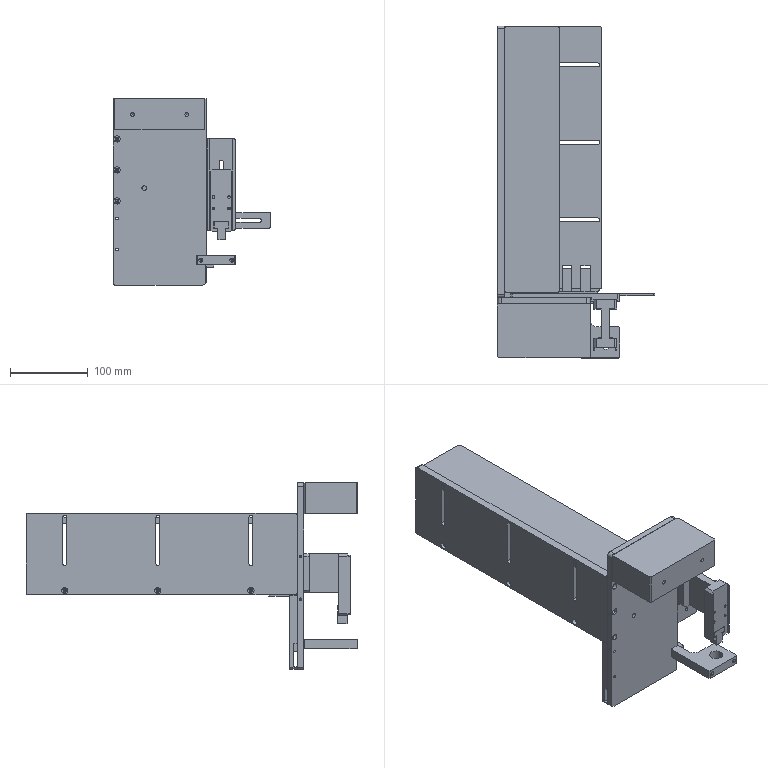Assembly | SolidWorks | mm | 13 component files | 13 solids | 410 faces | box 203.38 x 428 x 240 mm | volume 1719772 mm3 | plane 202 | cylinder 160 | cone 48 | commonest cylinder face diameters 5 x25 4.2 x20 3.3 x20 6 x16 8 x16 4.5 x16 4 x13 5.5 x10
Bill of materials:
SecondGenerationFour-sidedLabelingFeedingAdjustmentBaffle | 1 |  | Thin rectangular base plate with rounded corners carrying three evenly spaced rectangular ribs/blocks standing across its width; one block has a small cross hole in its end face.
SecondGenerationFour-sidedLabelingFeedingCylinderConnector | 1 |  | T-shaped block: wider rectangular head over a narrower rectangular stem, with a round through hole running vertically through the center.
SecondGenerationFour-sidedLabelingFeedingFrontBaffle | 1 |  | Long thin rectangular plate with three narrow slots running across its width, open at one long edge, plus a comb-like set of rectangular notches/fingers at one end; a small hole or slot is visible on one end edge.
SecondGenerationFour-sidedLabelingFeedingFrontLimitPlate | 1 |  | Long, slender rectangular bar with a shallow step at one end and a downturned rectangular block at the other end, forming an L/hook shape in side profile; a round hole goes through the end block.
SecondGenerationFour-sidedLabelingFeedingLimitPlate | 1 |  | Elongated rectangular bar with two round holes along its length and a reduced-thickness notched section near one end that ends in a small hook/lip.
SecondGenerationFour-sidedLabelingFeedingRearBaffle | 1 |  | Long thin rectangular plate with small rounded corners, two small tabs sticking out from one long edge, and a tapered/chamfered underside at one end.
SecondGenerationFour-sidedLabelingSideBaffle | 1 |  | Rectangular plate with rounded corners, three parallel elongated slots, a small hole in line with each slot, and small holes in one short edge face.
SecondGenerationFour-sidedLabelingTopBatteryPlate | 1 |  | Flat plate with rounded corners shaped like a rectangle with a tab extending down from one corner; it has one long slot and a small hole in the tab, and a stepped/thinner region on the tab side.
SecondGenerationFour-sidedLabelingTopBatterySidePlate | 1 |  | Thin, flat, rectangular strip with rounded corners and one long central slot with rounded ends running most of its length.
ThirdGenerationFeedingBasePlate | 1 |  | Rectangular flat plate with rounded corners and many small round holes of a few sizes, mostly near the edges, plus one hole nearer the middle.
ThirdGenerationFour-sidedLabelingCylinderFixingPlate | 1 |  | Thick L-shaped block with a filleted inside corner and small corner chamfers; a large round vertical through hole sits in the wider portion, and two smaller holes go into one side face.
ThirdGenerationFour-sidedLabelingFeedingSliderConnectionPlate | 1 |  | Complex block with an I-shaped top profile (flanges at both ends joined by a narrower web) and an L-shaped side profile; one end has a slot with an inward-facing lip, and several small holes/half-holes are present on the faces.
ThirdGenerationFour-sidedLabelingFeedingSupportPlate | 1 |  | Solid rectangular block with small chamfers on its four short vertical edges and two small round holes on one long side face. The holes look like blind drilled holes with cone-shaped bottoms.
Mates:
1. concentric | ThirdGenerationFour-sidedLabelingFeedingSupportPlate-1 face at (-70.027, 33.863, 12) dir (0, 1, 0) r 2.1 | ThirdGenerationFeedingBasePlate-1 face at (-70.027, 41.863, 12) dir (0, 1, 0) r 2.75
2. concentric | ThirdGenerationFour-sidedLabelingFeedingSupportPlate-1 face at (29.973, 33.863, 12) dir (0, 1, 0) r 2.1 | ThirdGenerationFeedingBasePlate-1 face at (29.973, 41.863, 12) dir (0, 1, 0) r 2.75
3. coincident | ThirdGenerationFour-sidedLabelingFeedingSupportPlate-1 face at (-80.027, 33.863, 20) dir (0, 1, 0) | ThirdGenerationFeedingBasePlate-1 face at (-80.027, 33.863, -220) dir (0, -1, 0)
4. coincident | SecondGenerationFour-sidedLabelingTopBatteryPlate-1 face at (7.473, 38.863, -79) dir (0, -1, 0) | ThirdGenerationFour-sidedLabelingFeedingSliderConnectionPlate-1 face at (44.473, 38.863, -71.5) dir (0, 1, 0)
5. coincident | SecondGenerationFour-sidedLabelingTopBatterySidePlate-1 face at (3.358, 43.863, -126.5) dir (0, -1, 0) | SecondGenerationFour-sidedLabelingTopBatteryPlate-1 face at (41.473, 43.863, -146.5) dir (0, 1, 0)
6. coincident | ThirdGenerationFour-sidedLabelingFeedingSliderConnectionPlate-1 face at (68.973, -26.137, -138.5) dir (-1, 0, 0) | SecondGenerationFour-sidedLabelingFeedingCylinderConnector-1 face at (68.973, -10.137, -138.5) dir (1, 0, 0)
7. coincident | ThirdGenerationFour-sidedLabelingFeedingSliderConnectionPlate-1 face at (68.973, -26.137, -146.5) dir (0, 0, 1) | SecondGenerationFour-sidedLabelingFeedingCylinderConnector-1 face at (50.973, -10.137, -146.5) dir (0, 0, -1)
8. coincident | SecondGenerationFour-sidedLabelingTopBatteryPlate-1 face at (77.473, 46.863, -126.5) dir (0, 0, -1) | SecondGenerationFour-sidedLabelingTopBatterySidePlate-1 face at (123.358, 46.863, -126.5) dir (0, 0, 1)
9. coincident | ThirdGenerationFour-sidedLabelingFeedingSupportPlate-1 face at (-80.027, -36.137, 20) dir (0, -1, 0) | ThirdGenerationFour-sidedLabelingCylinderFixingPlate-1 face at (27.973, -36.137, -182) dir (0, -1, 0)
10. coincident | ThirdGenerationFeedingBasePlate-1 face at (-80.027, 41.863, -220) dir (0, 1, 0) | SecondGenerationFour-sidedLabelingSideBaffle-1 face at (-70.027, 41.863, -19) dir (0, -1, 0)
11. coincident | SecondGenerationFour-sidedLabelingSideBaffle-1 face at (-70.027, 391.863, -19) dir (1, 0, 0) | SecondGenerationFour-sidedLabelingFeedingFrontBaffle-1 face at (-70.027, 391.863, -124) dir (-1, 0, 0)
12. coincident | SecondGenerationFour-sidedLabelingFeedingFrontBaffle-1 face at (54.973, 52.863, -124) dir (0, 0, -1) | SecondGenerationFour-sidedLabelingFeedingAdjustmentBaffle-1 face at (39.973, 36.495, -124) dir (0, 0, 1)
13. coincident | SecondGenerationFour-sidedLabelingFeedingFrontBaffle-1 face at (39.973, 82.863, -124) dir (-1, 0, 0) | SecondGenerationFour-sidedLabelingFeedingAdjustmentBaffle-1 face at (39.973, 90.439, -124) dir (1, 0, 0)
14. concentric | ThirdGenerationFeedingBasePlate-1 face at (33.973, 41.863, -188) dir (0, 1, 0) r 2.75 | ThirdGenerationFour-sidedLabelingCylinderFixingPlate-1 face at (33.973, 33.863, -188) dir (0, 1, 0) r 2.1
15. parallel | ThirdGenerationFeedingBasePlate-1 face at (39.973, 41.863, 20) dir (1, 0, 0) | ThirdGenerationFour-sidedLabelingFeedingSliderConnectionPlate-1 face at (44.473, -26.137, -151.5) dir (-1, 0, 0)
16. coincident | ThirdGenerationFeedingBasePlate-1 face at (-80.027, 41.863, -220) dir (0, 1, 0) | SecondGenerationFour-sidedLabelingFeedingLimitPlate-1 face at (-70.027, 41.863, -124) dir (0, -1, 0)
17. coincident | ThirdGenerationFeedingBasePlate-1 face at (-80.027, 41.863, -220) dir (0, 1, 0) | SecondGenerationFour-sidedLabelingFeedingFrontLimitPlate-1 face at (-70.027, 41.863, -187) dir (0, -1, 0)
18. coincident | ThirdGenerationFeedingBasePlate-1 face at (39.973, 41.863, 20) dir (1, 0, 0) | SecondGenerationFour-sidedLabelingFeedingFrontLimitPlate-1 face at (39.973, 33.863, -197) dir (-1, 0, 0)
19. coincident | SecondGenerationFour-sidedLabelingSideBaffle-1 face at (-70.027, 391.863, -19) dir (1, 0, 0) | SecondGenerationFour-sidedLabelingFeedingRearBaffle-1 face at (-70.027, 391.863, -24) dir (-1, 0, 0)
20. distance | SecondGenerationFour-sidedLabelingFeedingFrontLimitPlate-1 face at (-70.027, 51.863, -197) dir (0, 0, -1) | ThirdGenerationFeedingBasePlate-1 face at (39.973, 41.863, -220) dir (0, 0, -1)
21. coincident | ThirdGenerationFour-sidedLabelingFeedingSliderConnectionPlate-1 face at (74.473, -26.137, -151.5) dir (1, 0, 0) | SecondGenerationFour-sidedLabelingTopBatteryPlate-1 face at (74.473, 38.863, -31.5) dir (-1, 0, 0)
22. coincident | SecondGenerationFour-sidedLabelingFeedingLimitPlate-1 face at (-80.027, 51.863, -124) dir (0, 0, 1) | SecondGenerationFour-sidedLabelingSideBaffle-1 face at (-80.027, 391.863, -124) dir (0, 0, -1)
23. distance | SecondGenerationFour-sidedLabelingFeedingFrontBaffle-1 face at (54.973, 52.863, -114) dir (0, 0, 1) | SecondGenerationFour-sidedLabelingFeedingRearBaffle-1 face at (-0.02689, 46.863, -32) dir (0, 0, -1)
24. coincident | ThirdGenerationFeedingBasePlate-1 face at (39.973, 41.863, -220) dir (0, 0, -1) | SecondGenerationFour-sidedLabelingFeedingLimitPlate-1 face at (-80.027, 51.863, -220) dir (0, 0, -1)
25. coincident | ThirdGenerationFeedingBasePlate-1 face at (-80.027, 41.863, 20) dir (-1, 0, 0) | SecondGenerationFour-sidedLabelingFeedingLimitPlate-1 face at (-80.027, 51.863, -124) dir (-1, 0, 0)
26. coincident | ThirdGenerationFeedingBasePlate-1 face at (-80.027, 41.863, 20) dir (-1, 0, 0) | SecondGenerationFour-sidedLabelingSideBaffle-1 face at (-80.027, 391.863, -19) dir (-1, 0, 0)
27. distance | SecondGenerationFour-sidedLabelingTopBatteryPlate-1 face at (-62.527, 46.863, -31.5) dir (0, 1, 0) | SecondGenerationFour-sidedLabelingFeedingRearBaffle-1 face at (-108.841, 47.863, -32) dir (0, -1, 0)
28. coincident | SecondGenerationFour-sidedLabelingSideBaffle-1 face at (-80.027, 391.863, -124) dir (0, 0, -1) | SecondGenerationFour-sidedLabelingFeedingFrontBaffle-1 face at (54.973, 52.863, -124) dir (0, 0, -1)
29. distance | SecondGenerationFour-sidedLabelingFeedingFrontBaffle-1 face at (54.973, 52.863, -124) dir (0, -1, 0) | ThirdGenerationFeedingBasePlate-1 face at (-80.027, 41.863, -220) dir (0, 1, 0)